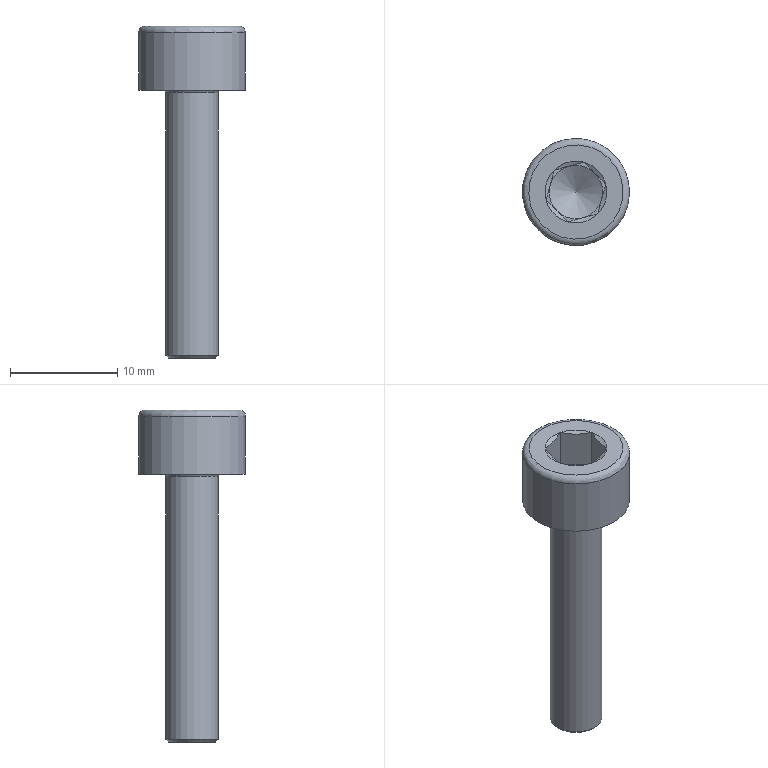Component | NX | SCREW_M6X25 | 1 solid | 27 faces | volume 848 mm3 | plane 15 | cone 8 | cylinder 2 | torus 2 | commonest cylinder face diameters 4.891 x1 10 x1